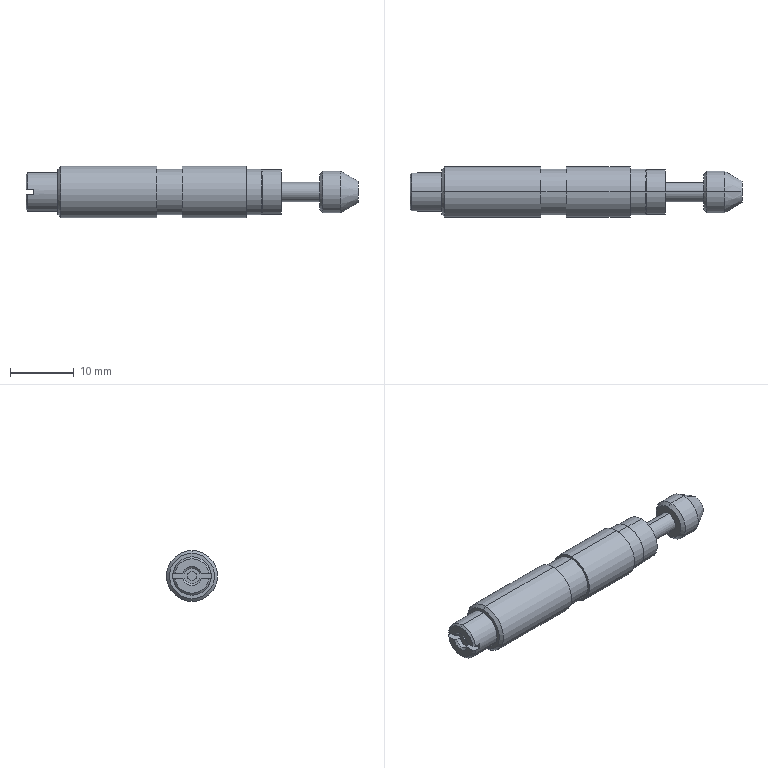Component | SolidWorks | CCDJSACA0806-1-2_CCDJSACA-0806-1_Body-1 | 1 solid | 55 faces | box 52 x 8 x 8 mm | volume 1991 mm3 | plane 22 | cylinder 18 | cone 15 | commonest cylinder face diameters 8 x4 7.188 x4 6 x2 7 x2 3 x2 6.5 x2 2.459 x2
build123d program:
from build123d import *

# Parameters (mm, degrees)
CUT_EXTRUDE1_DEPTH      = 2.5
CUT_EXTRUDE2_DEPTH      = 0.4
CUT_EXTRUDE2_DEPTH_BACK = 0.4
SKETCH4_W               = 8
SKETCH4_H               = 1.2
SKETCH1_W               = 1.006
SKETCH1_H               = 4
SKETCH1_H_2             = 3


with BuildPart() as part:
    # Sketch1_2 → Revolve1 (revolve)
    with BuildSketch(Plane.XY, mode=Mode.PRIVATE) as revolve1_sk:
        Polygon((0, 52), (1.71, 52), (3.25, 49.333), (3.25, 46.5), (2.75, 46), (1.5, 46), (1.5, 40), (3.5, 40), (3.5, 37), (3.54, 37), (4, 36.54), (4, 5.46), (3.54, 5), (3, 5), (3, 0.3), (2.7, 0), (0, 0), align=None)
    revolve(revolve1_sk.sketch.rotate(Axis((0, 0, 0), (0, 1, 0)), 270), axis=Axis((0, 0, 0), (0, 1, 0)))

    # Sketch2 → Cut-Revolve1_2 (revolve, cut)
    with BuildSketch(Plane.XY, mode=Mode.PRIVATE) as cut_revolve1_2_sk:
        Polygon((0, 1.2), (1.5, 1.2), (1.23, 0.9295), (1.23, 0.2705), (1.5, 0), (0, 0), align=None)
    revolve(cut_revolve1_2_sk.sketch.rotate(Axis((0, 0, 0), (0, 1, 0)), 180), axis=Axis((0, 0, 0), (0, 1, 0)), mode=Mode.SUBTRACT)

    # Sketch3 → Cut-Extrude1 (cut)
    with BuildSketch(Plane(origin=(0, 0, 0), x_dir=(1, 0, 0), z_dir=(0, 1, 0))):
        Polygon((-0.6495, -0.375), (0, -0.75), (0.6495, -0.375), (0.6495, 0.375), (0, 0.75), (-0.6495, 0.375), align=None)
    extrude(amount=CUT_EXTRUDE1_DEPTH, mode=Mode.SUBTRACT)

    # Sketch4 → Cut-Extrude2 (cut, two sides: drawn at the far end of the back side and taken through both)
    with BuildSketch(Plane.XY.offset(-CUT_EXTRUDE2_DEPTH_BACK)):
        with Locations((0, 0.6)):
            Rectangle(SKETCH4_W, SKETCH4_H)
    extrude(amount=CUT_EXTRUDE2_DEPTH + CUT_EXTRUDE2_DEPTH_BACK, mode=Mode.SUBTRACT)

    # Sketch1 → Cut-Revolve1 (revolve, cut)
    with BuildSketch(Plane.XY, mode=Mode.PRIVATE) as cut_revolve1_sk:
        with Locations((4.097, 22.5)):
            Rectangle(SKETCH1_W, SKETCH1_H)
        with Locations((4.097, 36)):
            Rectangle(SKETCH1_W, SKETCH1_H_2)
    revolve(cut_revolve1_sk.sketch.rotate(Axis((0, 19.5, 0), (0, 1, 0)), 90), axis=Axis((0, 19.5, 0), (0, 1, 0)), mode=Mode.SUBTRACT)


solid = part.part

# Placed as in the assembly
solid = solid.moved(Location((-242.5, 399.564, -63.5), (0, 0, -90)))